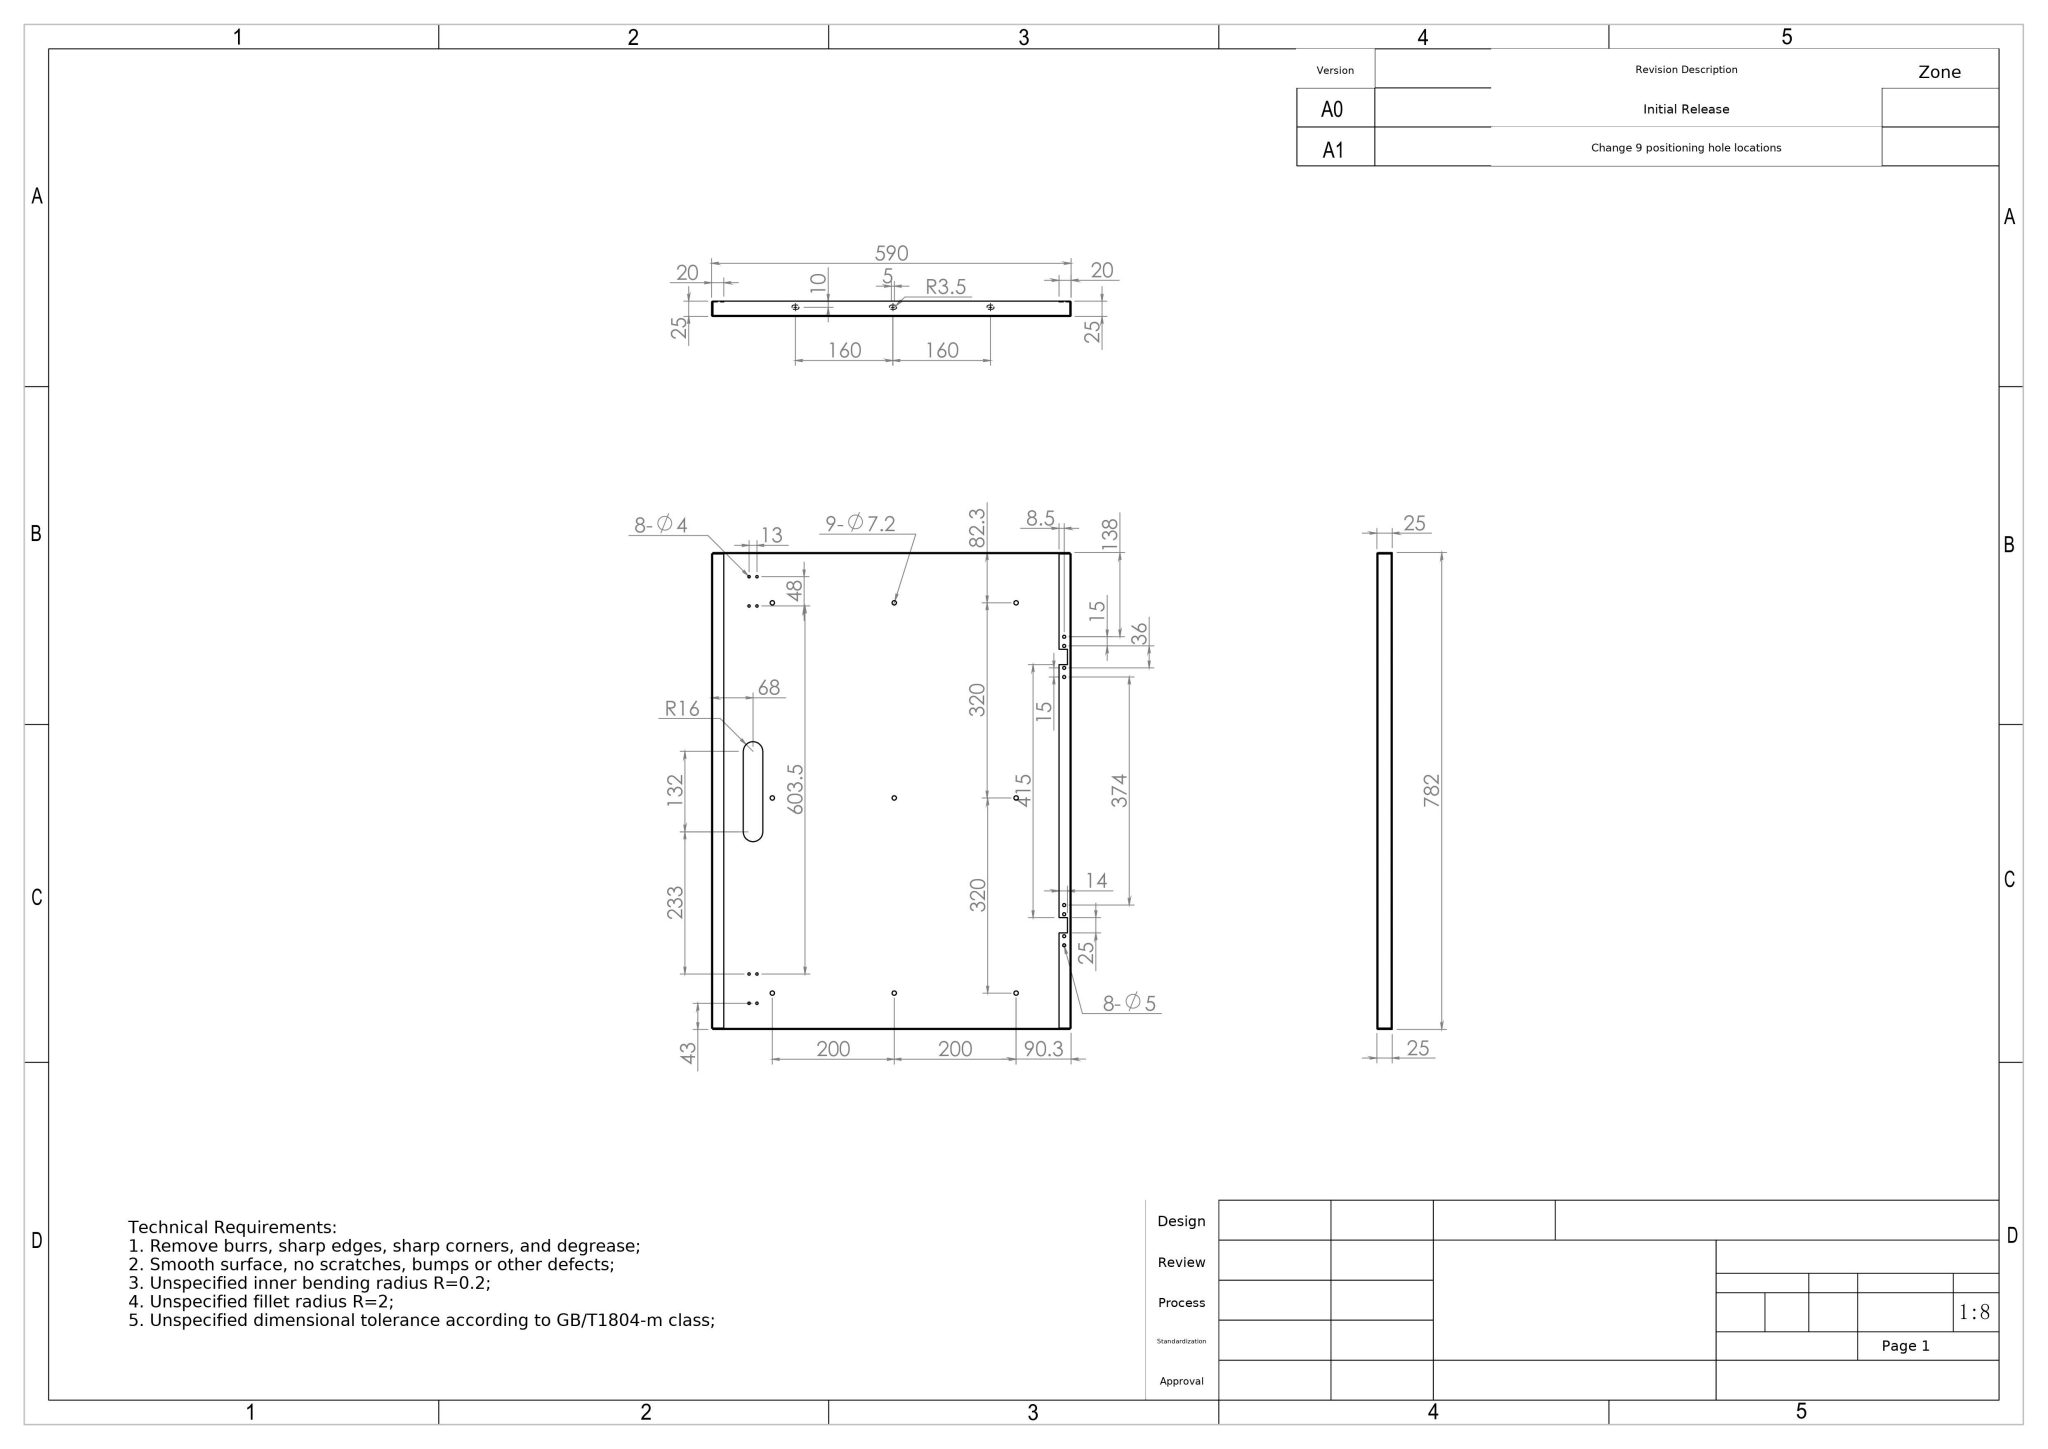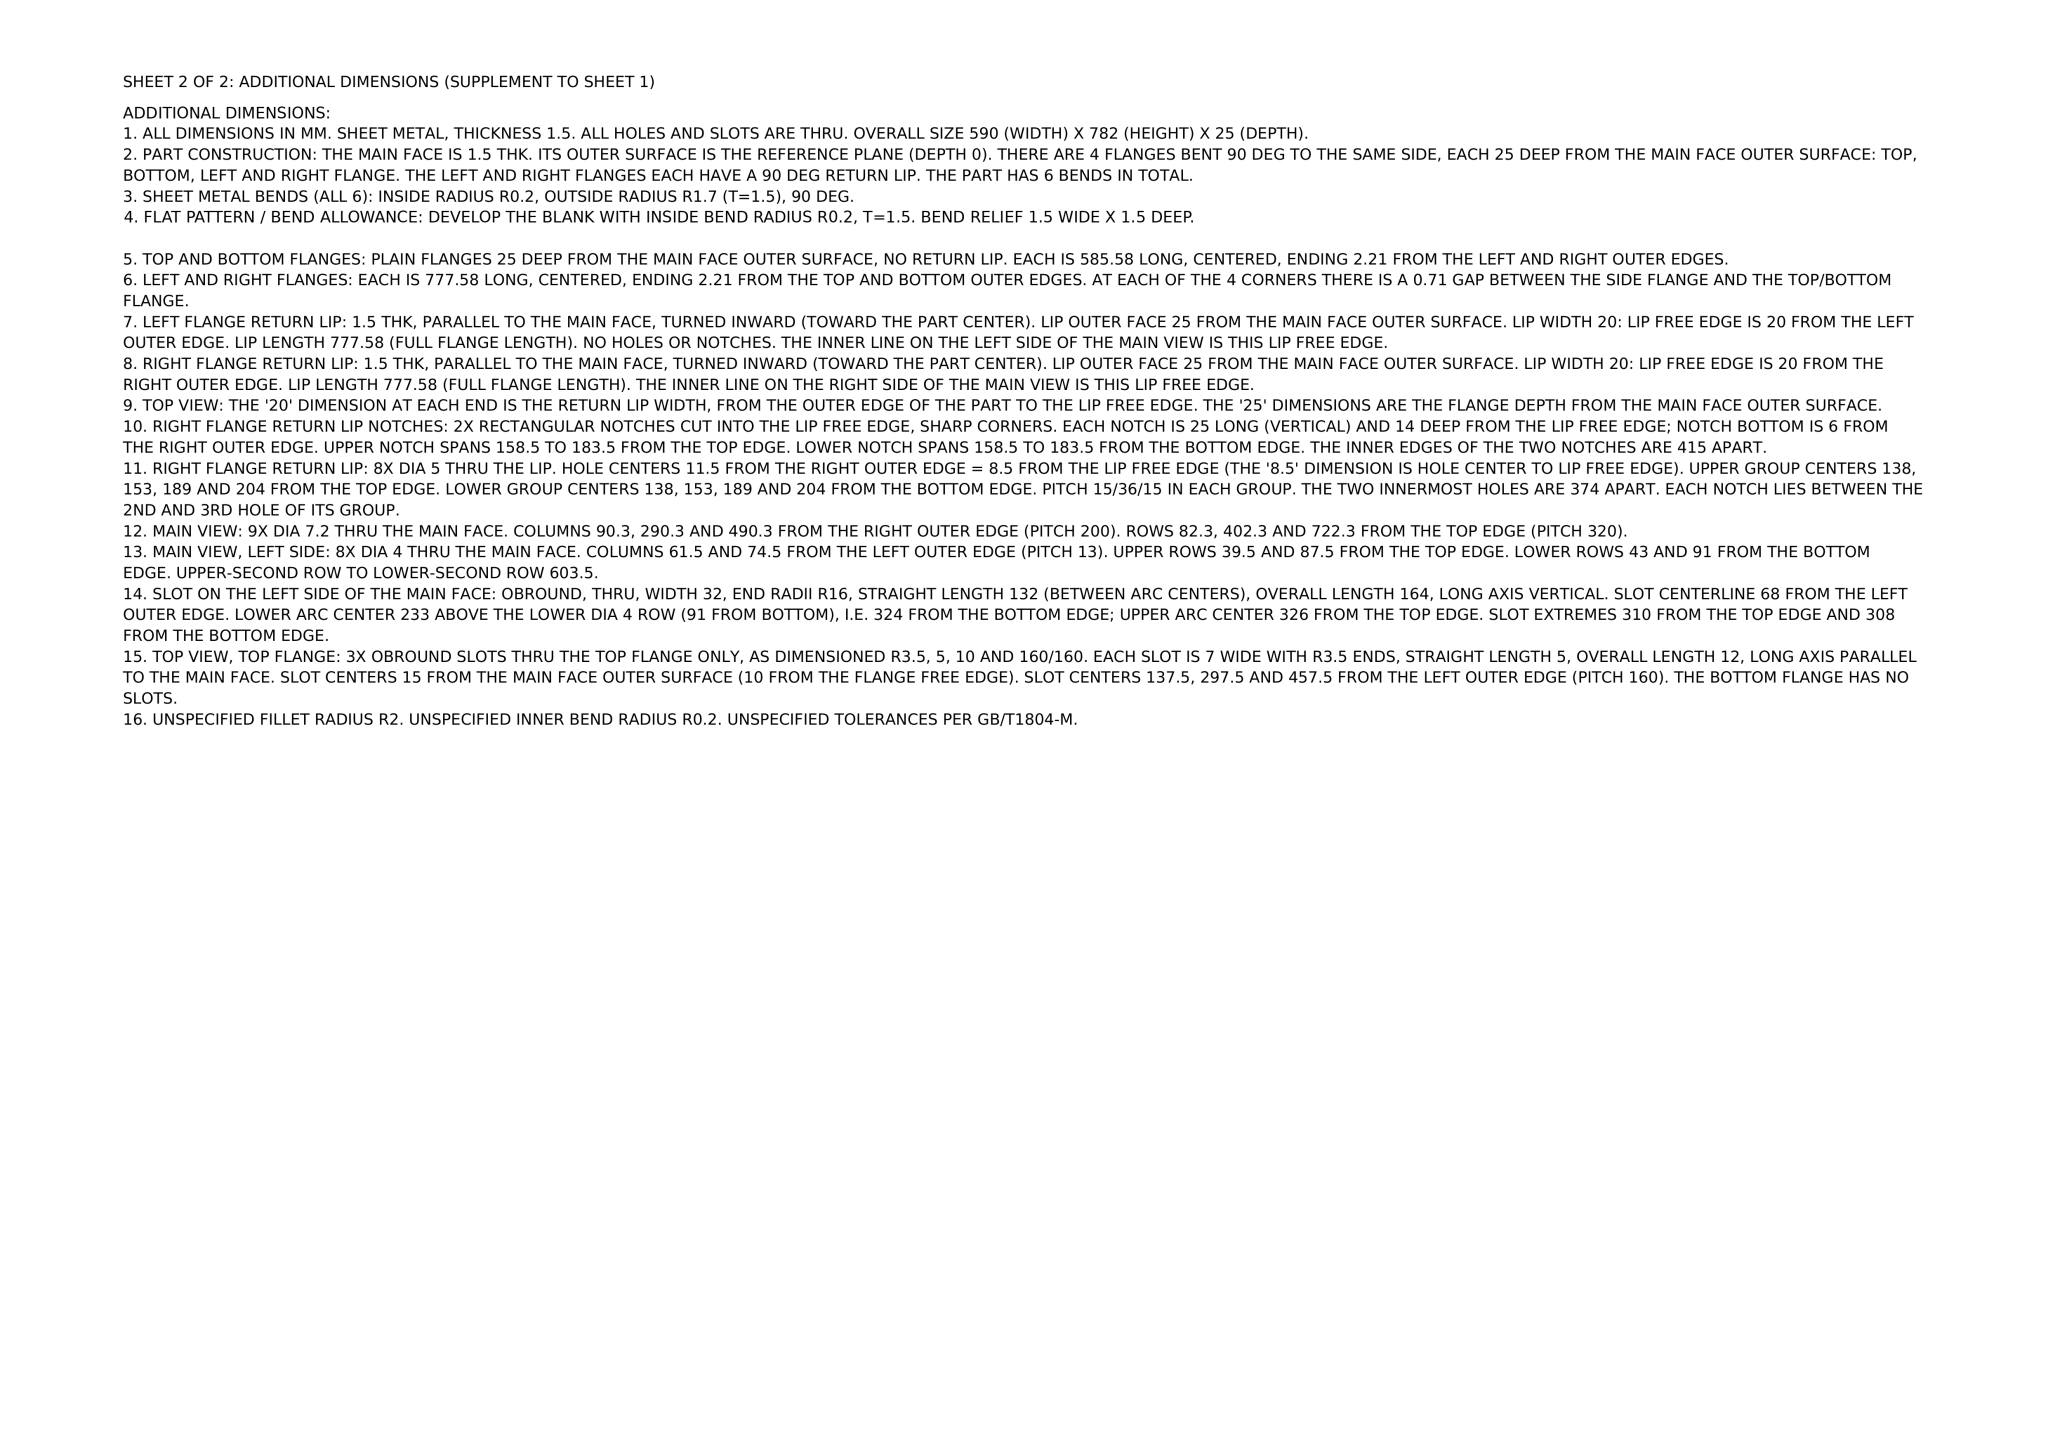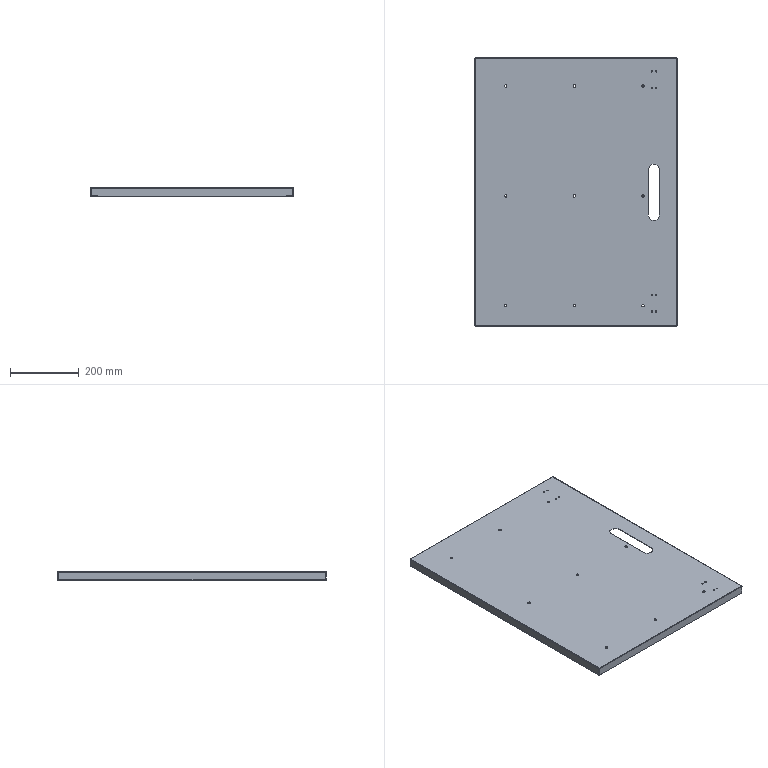Part | NX | mm | 1 solid | 128 faces | box 590 x 782 x 25 mm | volume 818829 mm3 | cylinder 70 | plane 50 | spline 8 | commonest cylinder face diameters 7.2 x18 4 x16 5 x16 3.4 x6 0.4 x6 7 x6 32 x2